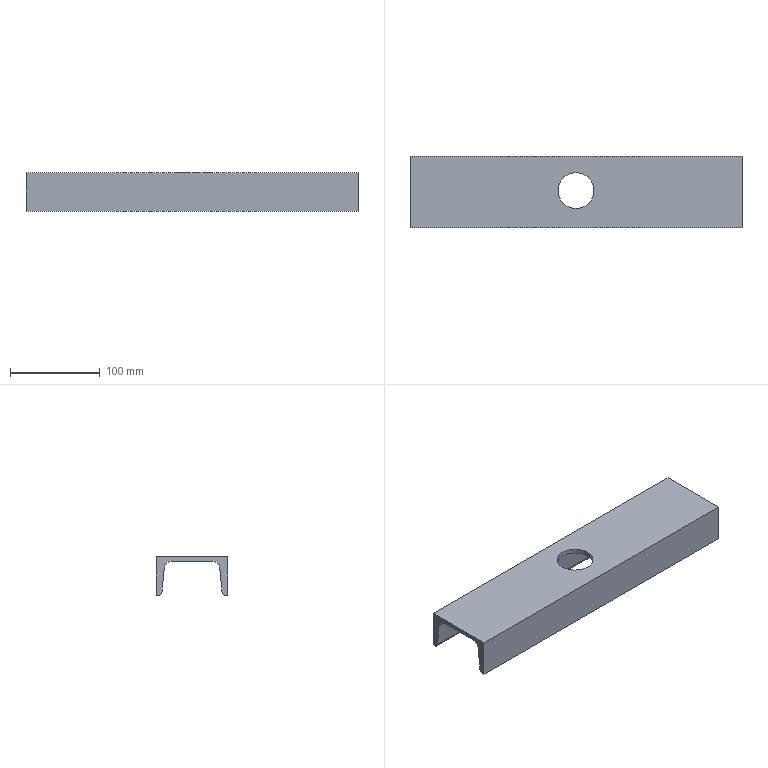Component | SolidWorks | ChannelSteelNo.8470-2-650-331Machine-1 | 1 solid | 16 faces | box 370 x 80 x 43 mm | volume 372695 mm3 | plane 10 | cylinder 6 | commonest cylinder face diameters 40 x2 16 x2 8 x2
build123d program:
from build123d import *

# Parameters (mm, degrees)
BOSS_EXTRUDE1_DEPTH = 370
SKETCH2_R           = 20
CUT_EXTRUDE1_DEPTH  = 381.984


with BuildPart() as part:
    # Sketch1 → Boss-Extrude1 (new body)
    with BuildSketch(Plane(origin=(0, 0, 0), x_dir=(-1, 0, 0), z_dir=(0, 0, -1))):
        with BuildLine():
            Line((-5, 62.86), (-5, 17.14))
            ThreePointArc((-5, 17.14), (-7.068, 11.772), (-12.204, 9.18))
            Line((-12.204, 9.18), (-39.398, 6.46))
            ThreePointArc((-39.398, 6.46), (-41.966, 5.164), (-43, 2.48))
            Line((-43, 2.48), (-43, 0))
            Line((-43, 0), (0, 0))
            Line((0, 0), (0, 80))
            Line((0, 80), (-43, 80))
            Line((-43, 80), (-43, 77.52))
            ThreePointArc((-43, 77.52), (-41.966, 74.836), (-39.398, 73.54))
            Line((-39.398, 73.54), (-12.204, 70.82))
            ThreePointArc((-12.204, 70.82), (-7.068, 68.228), (-5, 62.86))
        make_face()
    extrude(amount=-BOSS_EXTRUDE1_DEPTH)

    # Sketch2 → Cut-Extrude1 (cut, through all)
    with BuildSketch(Plane.ZY):
        with Locations((185, 41.5)):
            Circle(SKETCH2_R)
    extrude(amount=-CUT_EXTRUDE1_DEPTH, mode=Mode.SUBTRACT)


solid = part.part

# Placed as in the assembly
solid = solid.moved(Location((-286.681, 723.438, 647.223), (0, 90, 0)))
STEP:
#1=COLOUR_RGB('',0.7922,0.8196,0.9333);
#2=FILL_AREA_STYLE_COLOUR('',#1);
#3=FILL_AREA_STYLE('',(#2));
#4=SURFACE_STYLE_FILL_AREA(#3);
#5=SURFACE_SIDE_STYLE('',(#4));
#6=SURFACE_STYLE_USAGE(.BOTH.,#5);
#7=PRESENTATION_STYLE_ASSIGNMENT((#6));
#8=CARTESIAN_POINT('',(-3.216,30.116,25.284));
#9=VERTEX_POINT('',#8);
#10=CARTESIAN_POINT('',(-4.791,30.116,25.284));
#11=VERTEX_POINT('',#10);
#12=CARTESIAN_POINT('',(-4.003,30.116,25.284));
#13=DIRECTION('',(0.,0.,-1.));
#14=DIRECTION('',(0.,1.,0.));
#15=AXIS2_PLACEMENT_3D('',#12,#13,#14);
#16=CIRCLE('',#15,0.7874);
#17=EDGE_CURVE('',#9,#11,#16,.T.);
#18=ORIENTED_EDGE('',*,*,#17,.T.);
#19=CARTESIAN_POINT('',(-4.791,30.116,25.481));
#20=VERTEX_POINT('',#19);
#21=CARTESIAN_POINT('',(-4.791,30.116,23.788));
#22=DIRECTION('',(-0.,-0.,1.));
#23=VECTOR('',#22,39.37);
#24=LINE('',#21,#23);
#25=EDGE_CURVE('',#11,#20,#24,.T.);
#26=ORIENTED_EDGE('',*,*,#25,.T.);
#27=CARTESIAN_POINT('',(-3.216,30.116,25.481));
#28=VERTEX_POINT('',#27);
#29=CARTESIAN_POINT('',(-4.003,30.116,25.481));
#30=DIRECTION('',(-0.,-0.,1.));
#31=DIRECTION('',(1.,0.,0.));
#32=AXIS2_PLACEMENT_3D('',#29,#30,#31);
#33=CIRCLE('',#32,0.7874);
#34=EDGE_CURVE('',#20,#28,#33,.T.);
#35=ORIENTED_EDGE('',*,*,#34,.T.);
#36=CARTESIAN_POINT('',(-3.216,30.116,23.788));
#37=DIRECTION('',(-0.,-0.,1.));
#38=VECTOR('',#37,39.37);
#39=LINE('',#36,#38);
#40=EDGE_CURVE('',#9,#28,#39,.T.);
#41=ORIENTED_EDGE('',*,*,#40,.F.);
#42=EDGE_LOOP('',(#18,#26,#35,#41));
#43=FACE_OUTER_BOUND('',#42,.T.);
#44=CARTESIAN_POINT('',(-4.003,30.116,23.788));
#45=DIRECTION('',(-0.,-0.,1.));
#46=DIRECTION('',(1.,0.,0.));
#47=AXIS2_PLACEMENT_3D('',#44,#45,#46);
#48=CYLINDRICAL_SURFACE('',#47,0.7874);
#49=ADVANCED_FACE('',(#43),#48,.F.);
#50=CARTESIAN_POINT('',(-11.287,31.27,25.001));
#51=VERTEX_POINT('',#50);
#52=CARTESIAN_POINT('',(-11.287,30.957,25.284));
#53=VERTEX_POINT('',#52);
#54=CARTESIAN_POINT('',(-11.287,30.957,24.969));
#55=DIRECTION('',(1.,-0.,0.));
#56=DIRECTION('',(0.,0.,-1.));
#57=AXIS2_PLACEMENT_3D('',#54,#55,#56);
#58=CIRCLE('',#57,0.315);
#59=EDGE_CURVE('',#51,#53,#58,.T.);
#60=ORIENTED_EDGE('',*,*,#59,.F.);
#61=CARTESIAN_POINT('',(3.28,31.27,25.001));
#62=VERTEX_POINT('',#61);
#63=CARTESIAN_POINT('',(3.28,31.27,25.001));
#64=DIRECTION('',(-1.,0.,-0.));
#65=VECTOR('',#64,39.37);
#66=LINE('',#63,#65);
#67=EDGE_CURVE('',#62,#51,#66,.T.);
#68=ORIENTED_EDGE('',*,*,#67,.F.);
#69=CARTESIAN_POINT('',(3.28,30.957,25.284));
#70=VERTEX_POINT('',#69);
#71=CARTESIAN_POINT('',(3.28,30.957,24.969));
#72=DIRECTION('',(1.,-0.,0.));
#73=DIRECTION('',(0.,0.,-1.));
#74=AXIS2_PLACEMENT_3D('',#71,#72,#73);
#75=CIRCLE('',#74,0.315);
#76=EDGE_CURVE('',#62,#70,#75,.T.);
#77=ORIENTED_EDGE('',*,*,#76,.T.);
#78=CARTESIAN_POINT('',(3.28,30.957,25.284));
#79=DIRECTION('',(-1.,0.,-0.));
#80=VECTOR('',#79,39.37);
#81=LINE('',#78,#80);
#82=EDGE_CURVE('',#70,#53,#81,.T.);
#83=ORIENTED_EDGE('',*,*,#82,.T.);
#84=EDGE_LOOP('',(#60,#68,#77,#83));
#85=FACE_OUTER_BOUND('',#84,.T.);
#86=CARTESIAN_POINT('',(3.28,30.957,24.969));
#87=DIRECTION('',(-1.,0.,-0.));
#88=DIRECTION('',(0.,0.,1.));
#89=AXIS2_PLACEMENT_3D('',#86,#87,#88);
#90=CYLINDRICAL_SURFACE('',#89,0.315);
#91=ADVANCED_FACE('',(#85),#90,.F.);
#92=CARTESIAN_POINT('',(-11.287,31.377,23.93));
#93=VERTEX_POINT('',#92);
#94=CARTESIAN_POINT('',(-11.287,31.377,23.93));
#95=DIRECTION('',(-0.,-0.0995,0.995));
#96=VECTOR('',#95,39.37);
#97=LINE('',#94,#96);
#98=EDGE_CURVE('',#93,#51,#97,.T.);
#99=ORIENTED_EDGE('',*,*,#98,.F.);
#100=CARTESIAN_POINT('',(3.28,31.377,23.93));
#101=VERTEX_POINT('',#100);
#102=CARTESIAN_POINT('',(3.28,31.377,23.93));
#103=DIRECTION('',(-1.,0.,-0.));
#104=VECTOR('',#103,39.37);
#105=LINE('',#102,#104);
#106=EDGE_CURVE('',#101,#93,#105,.T.);
#107=ORIENTED_EDGE('',*,*,#106,.F.);
#108=CARTESIAN_POINT('',(3.28,31.377,23.93));
#109=DIRECTION('',(-0.,-0.0995,0.995));
#110=VECTOR('',#109,39.37);
#111=LINE('',#108,#110);
#112=EDGE_CURVE('',#101,#62,#111,.T.);
#113=ORIENTED_EDGE('',*,*,#112,.T.);
#114=ORIENTED_EDGE('',*,*,#67,.T.);
#115=EDGE_LOOP('',(#99,#107,#113,#114));
#116=FACE_OUTER_BOUND('',#115,.T.);
#117=CARTESIAN_POINT('',(3.28,31.377,23.93));
#118=DIRECTION('',(-0.,-0.995,-0.0995));
#119=DIRECTION('',(0.,0.0995,-0.995));
#120=AXIS2_PLACEMENT_3D('',#117,#118,#119);
#121=PLANE('',#120);
#122=ADVANCED_FACE('',(#116),#121,.T.);
#123=CARTESIAN_POINT('',(-11.287,31.534,23.788));
#124=VERTEX_POINT('',#123);
#125=CARTESIAN_POINT('',(-11.287,31.534,23.946));
#126=DIRECTION('',(-1.,0.,-0.));
#127=DIRECTION('',(0.,0.,1.));
#128=AXIS2_PLACEMENT_3D('',#125,#126,#127);
#129=CIRCLE('',#128,0.1575);
#130=EDGE_CURVE('',#124,#93,#129,.T.);
#131=ORIENTED_EDGE('',*,*,#130,.F.);
#132=CARTESIAN_POINT('',(3.28,31.534,23.788));
#133=VERTEX_POINT('',#132);
#134=CARTESIAN_POINT('',(3.28,31.534,23.788));
#135=DIRECTION('',(-1.,0.,-0.));
#136=VECTOR('',#135,39.37);
#137=LINE('',#134,#136);
#138=EDGE_CURVE('',#133,#124,#137,.T.);
#139=ORIENTED_EDGE('',*,*,#138,.F.);
#140=CARTESIAN_POINT('',(3.28,31.534,23.946));
#141=DIRECTION('',(-1.,0.,-0.));
#142=DIRECTION('',(0.,0.,1.));
#143=AXIS2_PLACEMENT_3D('',#140,#141,#142);
#144=CIRCLE('',#143,0.1575);
#145=EDGE_CURVE('',#133,#101,#144,.T.);
#146=ORIENTED_EDGE('',*,*,#145,.T.);
#147=ORIENTED_EDGE('',*,*,#106,.T.);
#148=EDGE_LOOP('',(#131,#139,#146,#147));
#149=FACE_OUTER_BOUND('',#148,.T.);
#150=CARTESIAN_POINT('',(3.28,31.534,23.946));
#151=DIRECTION('',(-1.,0.,-0.));
#152=DIRECTION('',(0.,0.,1.));
#153=AXIS2_PLACEMENT_3D('',#150,#151,#152);
#154=CYLINDRICAL_SURFACE('',#153,0.1575);
#155=ADVANCED_FACE('',(#149),#154,.T.);
#156=CARTESIAN_POINT('',(-11.287,31.631,23.788));
#157=VERTEX_POINT('',#156);
#158=CARTESIAN_POINT('',(-11.287,31.631,23.788));
#159=DIRECTION('',(-0.,-1.,-0.));
#160=VECTOR('',#159,39.37);
#161=LINE('',#158,#160);
#162=EDGE_CURVE('',#157,#124,#161,.T.);
#163=ORIENTED_EDGE('',*,*,#162,.F.);
#164=CARTESIAN_POINT('',(3.28,31.631,23.788));
#165=VERTEX_POINT('',#164);
#166=CARTESIAN_POINT('',(3.28,31.631,23.788));
#167=DIRECTION('',(-1.,0.,-0.));
#168=VECTOR('',#167,39.37);
#169=LINE('',#166,#168);
#170=EDGE_CURVE('',#165,#157,#169,.T.);
#171=ORIENTED_EDGE('',*,*,#170,.F.);
#172=CARTESIAN_POINT('',(3.28,31.631,23.788));
#173=DIRECTION('',(-0.,-1.,-0.));
#174=VECTOR('',#173,39.37);
#175=LINE('',#172,#174);
#176=EDGE_CURVE('',#165,#133,#175,.T.);
#177=ORIENTED_EDGE('',*,*,#176,.T.);
#178=ORIENTED_EDGE('',*,*,#138,.T.);
#179=EDGE_LOOP('',(#163,#171,#177,#178));
#180=FACE_OUTER_BOUND('',#179,.T.);
#181=CARTESIAN_POINT('',(3.28,31.631,23.788));
#182=DIRECTION('',(0.,0.,-1.));
#183=DIRECTION('',(-1.,0.,-0.));
#184=AXIS2_PLACEMENT_3D('',#181,#182,#183);
#185=PLANE('',#184);
#186=ADVANCED_FACE('',(#180),#185,.T.);
#187=CARTESIAN_POINT('',(-11.287,31.631,25.481));
#188=VERTEX_POINT('',#187);
#189=CARTESIAN_POINT('',(-11.287,31.631,25.481));
#190=DIRECTION('',(0.,0.,-1.));
#191=VECTOR('',#190,39.37);
#192=LINE('',#189,#191);
#193=EDGE_CURVE('',#188,#157,#192,.T.);
#194=ORIENTED_EDGE('',*,*,#193,.F.);
#195=CARTESIAN_POINT('',(3.28,31.631,25.481));
#196=VERTEX_POINT('',#195);
#197=CARTESIAN_POINT('',(3.28,31.631,25.481));
#198=DIRECTION('',(-1.,0.,-0.));
#199=VECTOR('',#198,39.37);
#200=LINE('',#197,#199);
#201=EDGE_CURVE('',#196,#188,#200,.T.);
#202=ORIENTED_EDGE('',*,*,#201,.F.);
#203=CARTESIAN_POINT('',(3.28,31.631,25.481));
#204=DIRECTION('',(0.,0.,-1.));
#205=VECTOR('',#204,39.37);
#206=LINE('',#203,#205);
#207=EDGE_CURVE('',#196,#165,#206,.T.);
#208=ORIENTED_EDGE('',*,*,#207,.T.);
#209=ORIENTED_EDGE('',*,*,#170,.T.);
#210=EDGE_LOOP('',(#194,#202,#208,#209));
#211=FACE_OUTER_BOUND('',#210,.T.);
#212=CARTESIAN_POINT('',(3.28,31.631,25.481));
#213=DIRECTION('',(0.,1.,0.));
#214=DIRECTION('',(1.,-0.,0.));
#215=AXIS2_PLACEMENT_3D('',#212,#213,#214);
#216=PLANE('',#215);
#217=ADVANCED_FACE('',(#211),#216,.T.);
#218=CARTESIAN_POINT('',(-4.003,30.116,25.481));
#219=DIRECTION('',(-0.,-0.,1.));
#220=DIRECTION('',(1.,0.,0.));
#221=AXIS2_PLACEMENT_3D('',#218,#219,#220);
#222=CIRCLE('',#221,0.7874);
#223=EDGE_CURVE('',#28,#20,#222,.T.);
#224=ORIENTED_EDGE('',*,*,#223,.F.);
#225=ORIENTED_EDGE('',*,*,#34,.F.);
#226=EDGE_LOOP('',(#224,#225));
#227=FACE_BOUND('',#226,.T.);
#228=CARTESIAN_POINT('',(-11.287,28.482,25.481));
#229=VERTEX_POINT('',#228);
#230=CARTESIAN_POINT('',(-11.287,28.482,25.481));
#231=DIRECTION('',(0.,1.,0.));
#232=VECTOR('',#231,39.37);
#233=LINE('',#230,#232);
#234=EDGE_CURVE('',#229,#188,#233,.T.);
#235=ORIENTED_EDGE('',*,*,#234,.F.);
#236=CARTESIAN_POINT('',(3.28,28.482,25.481));
#237=VERTEX_POINT('',#236);
#238=CARTESIAN_POINT('',(3.28,28.482,25.481));
#239=DIRECTION('',(-1.,0.,-0.));
#240=VECTOR('',#239,39.37);
#241=LINE('',#238,#240);
#242=EDGE_CURVE('',#237,#229,#241,.T.);
#243=ORIENTED_EDGE('',*,*,#242,.F.);
#244=CARTESIAN_POINT('',(3.28,28.482,25.481));
#245=DIRECTION('',(0.,1.,0.));
#246=VECTOR('',#245,39.37);
#247=LINE('',#244,#246);
#248=EDGE_CURVE('',#237,#196,#247,.T.);
#249=ORIENTED_EDGE('',*,*,#248,.T.);
#250=ORIENTED_EDGE('',*,*,#201,.T.);
#251=EDGE_LOOP('',(#235,#243,#249,#250));
#252=FACE_OUTER_BOUND('',#251,.T.);
#253=CARTESIAN_POINT('',(3.28,28.482,25.481));
#254=DIRECTION('',(-0.,-0.,1.));
#255=DIRECTION('',(1.,-0.,0.));
#256=AXIS2_PLACEMENT_3D('',#253,#254,#255);
#257=PLANE('',#256);
#258=ADVANCED_FACE('',(#227,#252),#257,.T.);
#259=CARTESIAN_POINT('',(-11.287,28.482,23.788));
#260=VERTEX_POINT('',#259);
#261=CARTESIAN_POINT('',(-11.287,28.482,23.788));
#262=DIRECTION('',(-0.,-0.,1.));
#263=VECTOR('',#262,39.37);
#264=LINE('',#261,#263);
#265=EDGE_CURVE('',#260,#229,#264,.T.);
#266=ORIENTED_EDGE('',*,*,#265,.F.);
#267=CARTESIAN_POINT('',(3.28,28.482,23.788));
#268=VERTEX_POINT('',#267);
#269=CARTESIAN_POINT('',(3.28,28.482,23.788));
#270=DIRECTION('',(-1.,0.,-0.));
#271=VECTOR('',#270,39.37);
#272=LINE('',#269,#271);
#273=EDGE_CURVE('',#268,#260,#272,.T.);
#274=ORIENTED_EDGE('',*,*,#273,.F.);
#275=CARTESIAN_POINT('',(3.28,28.482,23.788));
#276=DIRECTION('',(-0.,-0.,1.));
#277=VECTOR('',#276,39.37);
#278=LINE('',#275,#277);
#279=EDGE_CURVE('',#268,#237,#278,.T.);
#280=ORIENTED_EDGE('',*,*,#279,.T.);
#281=ORIENTED_EDGE('',*,*,#242,.T.);
#282=EDGE_LOOP('',(#266,#274,#280,#281));
#283=FACE_OUTER_BOUND('',#282,.T.);
#284=CARTESIAN_POINT('',(3.28,28.482,23.788));
#285=DIRECTION('',(-0.,-1.,-0.));
#286=DIRECTION('',(-1.,0.,-0.));
#287=AXIS2_PLACEMENT_3D('',#284,#285,#286);
#288=PLANE('',#287);
#289=ADVANCED_FACE('',(#283),#288,.T.);
#290=CARTESIAN_POINT('',(-11.287,28.579,23.788));
#291=VERTEX_POINT('',#290);
#292=CARTESIAN_POINT('',(-11.287,28.579,23.788));
#293=DIRECTION('',(-0.,-1.,-0.));
#294=VECTOR('',#293,39.37);
#295=LINE('',#292,#294);
#296=EDGE_CURVE('',#291,#260,#295,.T.);
#297=ORIENTED_EDGE('',*,*,#296,.F.);
#298=CARTESIAN_POINT('',(3.28,28.579,23.788));
#299=VERTEX_POINT('',#298);
#300=CARTESIAN_POINT('',(3.28,28.579,23.788));
#301=DIRECTION('',(-1.,0.,-0.));
#302=VECTOR('',#301,39.37);
#303=LINE('',#300,#302);
#304=EDGE_CURVE('',#299,#291,#303,.T.);
#305=ORIENTED_EDGE('',*,*,#304,.F.);
#306=CARTESIAN_POINT('',(3.28,28.579,23.788));
#307=DIRECTION('',(-0.,-1.,-0.));
#308=VECTOR('',#307,39.37);
#309=LINE('',#306,#308);
#310=EDGE_CURVE('',#299,#268,#309,.T.);
#311=ORIENTED_EDGE('',*,*,#310,.T.);
#312=ORIENTED_EDGE('',*,*,#273,.T.);
#313=EDGE_LOOP('',(#297,#305,#311,#312));
#314=FACE_OUTER_BOUND('',#313,.T.);
#315=CARTESIAN_POINT('',(3.28,28.579,23.788));
#316=DIRECTION('',(0.,0.,-1.));
#317=DIRECTION('',(0.,1.,0.));
#318=AXIS2_PLACEMENT_3D('',#315,#316,#317);
#319=PLANE('',#318);
#320=ADVANCED_FACE('',(#314),#319,.T.);
#321=CARTESIAN_POINT('',(-11.287,28.736,23.93));
#322=VERTEX_POINT('',#321);
#323=CARTESIAN_POINT('',(-11.287,28.579,23.946));
#324=DIRECTION('',(-1.,0.,-0.));
#325=DIRECTION('',(0.,0.,1.));
#326=AXIS2_PLACEMENT_3D('',#323,#324,#325);
#327=CIRCLE('',#326,0.1575);
#328=EDGE_CURVE('',#322,#291,#327,.T.);
#329=ORIENTED_EDGE('',*,*,#328,.F.);
#330=CARTESIAN_POINT('',(3.28,28.736,23.93));
#331=VERTEX_POINT('',#330);
#332=CARTESIAN_POINT('',(3.28,28.736,23.93));
#333=DIRECTION('',(-1.,0.,-0.));
#334=VECTOR('',#333,39.37);
#335=LINE('',#332,#334);
#336=EDGE_CURVE('',#331,#322,#335,.T.);
#337=ORIENTED_EDGE('',*,*,#336,.F.);
#338=CARTESIAN_POINT('',(3.28,28.579,23.946));
#339=DIRECTION('',(-1.,0.,-0.));
#340=DIRECTION('',(0.,0.,1.));
#341=AXIS2_PLACEMENT_3D('',#338,#339,#340);
#342=CIRCLE('',#341,0.1575);
#343=EDGE_CURVE('',#331,#299,#342,.T.);
#344=ORIENTED_EDGE('',*,*,#343,.T.);
#345=ORIENTED_EDGE('',*,*,#304,.T.);
#346=EDGE_LOOP('',(#329,#337,#344,#345));
#347=FACE_OUTER_BOUND('',#346,.T.);
#348=CARTESIAN_POINT('',(3.28,28.579,23.946));
#349=DIRECTION('',(-1.,0.,-0.));
#350=DIRECTION('',(0.,0.,1.));
#351=AXIS2_PLACEMENT_3D('',#348,#349,#350);
#352=CYLINDRICAL_SURFACE('',#351,0.1575);
#353=ADVANCED_FACE('',(#347),#352,.T.);
#354=CARTESIAN_POINT('',(-11.287,28.843,25.001));
#355=VERTEX_POINT('',#354);
#356=CARTESIAN_POINT('',(-11.287,28.843,25.001));
#357=DIRECTION('',(0.,-0.0995,-0.995));
#358=VECTOR('',#357,39.37);
#359=LINE('',#356,#358);
#360=EDGE_CURVE('',#355,#322,#359,.T.);
#361=ORIENTED_EDGE('',*,*,#360,.F.);
#362=CARTESIAN_POINT('',(3.28,28.843,25.001));
#363=VERTEX_POINT('',#362);
#364=CARTESIAN_POINT('',(3.28,28.843,25.001));
#365=DIRECTION('',(-1.,0.,-0.));
#366=VECTOR('',#365,39.37);
#367=LINE('',#364,#366);
#368=EDGE_CURVE('',#363,#355,#367,.T.);
#369=ORIENTED_EDGE('',*,*,#368,.F.);
#370=CARTESIAN_POINT('',(3.28,28.843,25.001));
#371=DIRECTION('',(0.,-0.0995,-0.995));
#372=VECTOR('',#371,39.37);
#373=LINE('',#370,#372);
#374=EDGE_CURVE('',#363,#331,#373,.T.);
#375=ORIENTED_EDGE('',*,*,#374,.T.);
#376=ORIENTED_EDGE('',*,*,#336,.T.);
#377=EDGE_LOOP('',(#361,#369,#375,#376));
#378=FACE_OUTER_BOUND('',#377,.T.);
#379=CARTESIAN_POINT('',(3.28,28.843,25.001));
#380=DIRECTION('',(0.,0.995,-0.0995));
#381=DIRECTION('',(-0.,0.0995,0.995));
#382=AXIS2_PLACEMENT_3D('',#379,#380,#381);
#383=PLANE('',#382);
#384=ADVANCED_FACE('',(#378),#383,.T.);
#385=CARTESIAN_POINT('',(-11.287,29.157,25.284));
#386=VERTEX_POINT('',#385);
#387=CARTESIAN_POINT('',(-11.287,29.157,24.969));
#388=DIRECTION('',(1.,-0.,0.));
#389=DIRECTION('',(0.,0.,-1.));
#390=AXIS2_PLACEMENT_3D('',#387,#388,#389);
#391=CIRCLE('',#390,0.315);
#392=EDGE_CURVE('',#386,#355,#391,.T.);
#393=ORIENTED_EDGE('',*,*,#392,.F.);
#394=CARTESIAN_POINT('',(3.28,29.157,25.284));
#395=VERTEX_POINT('',#394);
#396=CARTESIAN_POINT('',(3.28,29.157,25.284));
#397=DIRECTION('',(-1.,0.,-0.));
#398=VECTOR('',#397,39.37);
#399=LINE('',#396,#398);
#400=EDGE_CURVE('',#395,#386,#399,.T.);
#401=ORIENTED_EDGE('',*,*,#400,.F.);
#402=CARTESIAN_POINT('',(3.28,29.157,24.969));
#403=DIRECTION('',(1.,-0.,0.));
#404=DIRECTION('',(0.,0.,-1.));
#405=AXIS2_PLACEMENT_3D('',#402,#403,#404);
#406=CIRCLE('',#405,0.315);
#407=EDGE_CURVE('',#395,#363,#406,.T.);
#408=ORIENTED_EDGE('',*,*,#407,.T.);
#409=ORIENTED_EDGE('',*,*,#368,.T.);
#410=EDGE_LOOP('',(#393,#401,#408,#409));
#411=FACE_OUTER_BOUND('',#410,.T.);
#412=CARTESIAN_POINT('',(3.28,29.157,24.969));
#413=DIRECTION('',(-1.,0.,-0.));
#414=DIRECTION('',(0.,0.,1.));
#415=AXIS2_PLACEMENT_3D('',#412,#413,#414);
#416=CYLINDRICAL_SURFACE('',#415,0.315);
#417=ADVANCED_FACE('',(#411),#416,.F.);
#418=ORIENTED_EDGE('',*,*,#17,.F.);
#419=CARTESIAN_POINT('',(-4.003,30.116,25.284));
#420=DIRECTION('',(0.,0.,-1.));
#421=DIRECTION('',(0.,1.,0.));
#422=AXIS2_PLACEMENT_3D('',#419,#420,#421);
#423=CIRCLE('',#422,0.7874);
#424=EDGE_CURVE('',#11,#9,#423,.T.);
#425=ORIENTED_EDGE('',*,*,#424,.F.);
#426=EDGE_LOOP('',(#418,#425));
#427=FACE_BOUND('',#426,.T.);
#428=CARTESIAN_POINT('',(-11.287,30.957,25.284));
#429=DIRECTION('',(-0.,-1.,-0.));
#430=VECTOR('',#429,39.37);
#431=LINE('',#428,#430);
#432=EDGE_CURVE('',#53,#386,#431,.T.);
#433=ORIENTED_EDGE('',*,*,#432,.F.);
#434=ORIENTED_EDGE('',*,*,#82,.F.);
#435=CARTESIAN_POINT('',(3.28,30.957,25.284));
#436=DIRECTION('',(-0.,-1.,-0.));
#437=VECTOR('',#436,39.37);
#438=LINE('',#435,#437);
#439=EDGE_CURVE('',#70,#395,#438,.T.);
#440=ORIENTED_EDGE('',*,*,#439,.T.);
#441=ORIENTED_EDGE('',*,*,#400,.T.);
#442=EDGE_LOOP('',(#433,#434,#440,#441));
#443=FACE_OUTER_BOUND('',#442,.T.);
#444=CARTESIAN_POINT('',(3.28,30.957,25.284));
#445=DIRECTION('',(0.,0.,-1.));
#446=DIRECTION('',(0.,1.,0.));
#447=AXIS2_PLACEMENT_3D('',#444,#445,#446);
#448=PLANE('',#447);
#449=ADVANCED_FACE('',(#427,#443),#448,.T.);
#450=ORIENTED_EDGE('',*,*,#76,.F.);
#451=ORIENTED_EDGE('',*,*,#112,.F.);
#452=ORIENTED_EDGE('',*,*,#145,.F.);
#453=ORIENTED_EDGE('',*,*,#176,.F.);
#454=ORIENTED_EDGE('',*,*,#207,.F.);
#455=ORIENTED_EDGE('',*,*,#248,.F.);
#456=ORIENTED_EDGE('',*,*,#279,.F.);
#457=ORIENTED_EDGE('',*,*,#310,.F.);
#458=ORIENTED_EDGE('',*,*,#343,.F.);
#459=ORIENTED_EDGE('',*,*,#374,.F.);
#460=ORIENTED_EDGE('',*,*,#407,.F.);
#461=ORIENTED_EDGE('',*,*,#439,.F.);
#462=EDGE_LOOP('',(#450,#451,#452,#453,#454,#455,#456,#457,#458,#459,#460,#461));
#463=FACE_OUTER_BOUND('',#462,.T.);
#464=CARTESIAN_POINT('',(3.28,30.957,24.969));
#465=DIRECTION('',(1.,-0.,0.));
#466=DIRECTION('',(0.,0.,-1.));
#467=AXIS2_PLACEMENT_3D('',#464,#465,#466);
#468=PLANE('',#467);
#469=ADVANCED_FACE('',(#463),#468,.T.);
#470=ORIENTED_EDGE('',*,*,#59,.T.);
#471=ORIENTED_EDGE('',*,*,#432,.T.);
#472=ORIENTED_EDGE('',*,*,#392,.T.);
#473=ORIENTED_EDGE('',*,*,#360,.T.);
#474=ORIENTED_EDGE('',*,*,#328,.T.);
#475=ORIENTED_EDGE('',*,*,#296,.T.);
#476=ORIENTED_EDGE('',*,*,#265,.T.);
#477=ORIENTED_EDGE('',*,*,#234,.T.);
#478=ORIENTED_EDGE('',*,*,#193,.T.);
#479=ORIENTED_EDGE('',*,*,#162,.T.);
#480=ORIENTED_EDGE('',*,*,#130,.T.);
#481=ORIENTED_EDGE('',*,*,#98,.T.);
#482=EDGE_LOOP('',(#470,#471,#472,#473,#474,#475,#476,#477,#478,#479,#480,#481));
#483=FACE_OUTER_BOUND('',#482,.T.);
#484=CARTESIAN_POINT('',(-11.287,30.957,24.969));
#485=DIRECTION('',(1.,-0.,0.));
#486=DIRECTION('',(0.,0.,-1.));
#487=AXIS2_PLACEMENT_3D('',#484,#485,#486);
#488=PLANE('',#487);
#489=ADVANCED_FACE('',(#483),#488,.F.);
#490=ORIENTED_EDGE('',*,*,#25,.F.);
#491=ORIENTED_EDGE('',*,*,#424,.T.);
#492=ORIENTED_EDGE('',*,*,#40,.T.);
#493=ORIENTED_EDGE('',*,*,#223,.T.);
#494=EDGE_LOOP('',(#490,#491,#492,#493));
#495=FACE_OUTER_BOUND('',#494,.T.);
#496=CARTESIAN_POINT('',(-4.003,30.116,23.788));
#497=DIRECTION('',(-0.,-0.,1.));
#498=DIRECTION('',(1.,0.,0.));
#499=AXIS2_PLACEMENT_3D('',#496,#497,#498);
#500=CYLINDRICAL_SURFACE('',#499,0.7874);
#501=ADVANCED_FACE('',(#495),#500,.F.);
#502=CLOSED_SHELL('',(#49,#91,#122,#155,#186,#217,#258,#289,#320,#353,#384,#417,#449,#469,#489,#501));
#503=MANIFOLD_SOLID_BREP('',#502);
#504=STYLED_ITEM('',(#7),#503);
#505=(LENGTH_UNIT()NAMED_UNIT(*)SI_UNIT($,.METRE.));
#506=LENGTH_MEASURE_WITH_UNIT(LENGTH_MEASURE(0.0254),#505);
#507=DIMENSIONAL_EXPONENTS(1.,0.,0.,0.,0.,0.,0.);
#508=(CONVERSION_BASED_UNIT('',#506)LENGTH_UNIT()NAMED_UNIT(#507));
#509=UNCERTAINTY_MEASURE_WITH_UNIT(LENGTH_MEASURE(0.00001),#508,'','');
#510=(NAMED_UNIT(*)PLANE_ANGLE_UNIT()SI_UNIT($,.RADIAN.));
#511=(NAMED_UNIT(*)SI_UNIT($,.STERADIAN.)SOLID_ANGLE_UNIT());
#512=(GEOMETRIC_REPRESENTATION_CONTEXT(3)GLOBAL_UNCERTAINTY_ASSIGNED_CONTEXT((#509))GLOBAL_UNIT_ASSIGNED_CONTEXT((#508,#510,#511))REPRESENTATION_CONTEXT('',''));
#513=MECHANICAL_DESIGN_GEOMETRIC_PRESENTATION_REPRESENTATION('',(#504),#512);
#514=CARTESIAN_POINT('',(0.,0.,0.));
#515=DIRECTION('',(0.,0.,1.));
#516=DIRECTION('',(1.,0.,0.));
#517=AXIS2_PLACEMENT_3D('',#514,#515,#516);
#518=(LENGTH_UNIT()NAMED_UNIT(*)SI_UNIT($,.METRE.));
#519=LENGTH_MEASURE_WITH_UNIT(LENGTH_MEASURE(0.0254),#518);
#520=DIMENSIONAL_EXPONENTS(1.,0.,0.,0.,0.,0.,0.);
#521=(CONVERSION_BASED_UNIT('',#519)LENGTH_UNIT()NAMED_UNIT(#520));
#522=UNCERTAINTY_MEASURE_WITH_UNIT(LENGTH_MEASURE(0.00001),#521,'','');
#523=(NAMED_UNIT(*)PLANE_ANGLE_UNIT()SI_UNIT($,.RADIAN.));
#524=(NAMED_UNIT(*)SI_UNIT($,.STERADIAN.)SOLID_ANGLE_UNIT());
#525=(GEOMETRIC_REPRESENTATION_CONTEXT(3)GLOBAL_UNCERTAINTY_ASSIGNED_CONTEXT((#522))GLOBAL_UNIT_ASSIGNED_CONTEXT((#521,#523,#524))REPRESENTATION_CONTEXT('',''));
#526=ADVANCED_BREP_SHAPE_REPRESENTATION('',(#503,#517),#525);
#527=PRESENTATION_LAYER_ASSIGNMENT('','',(#504));